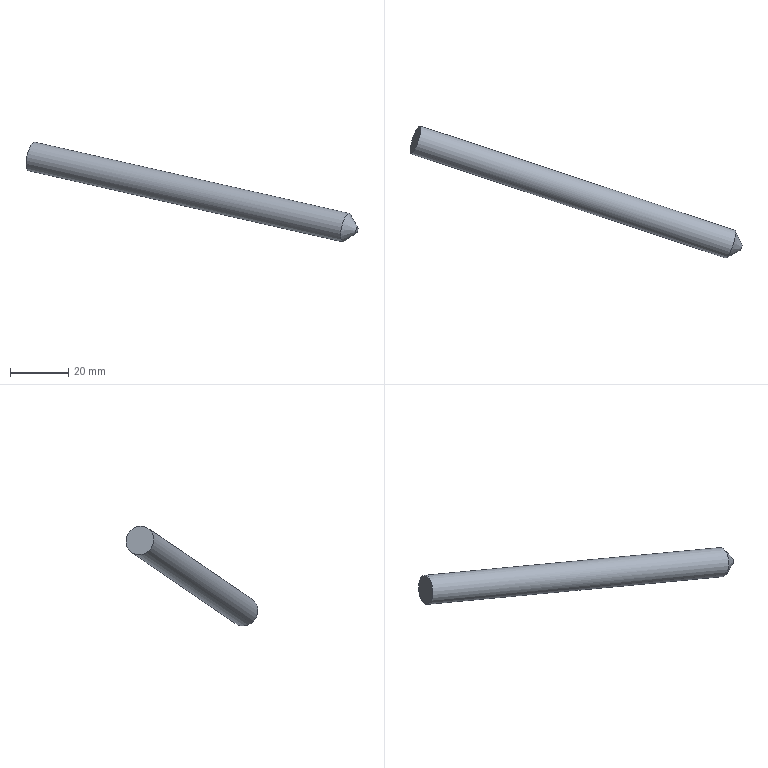Component | NX | PEN | 1 solid | 4 faces | box 113.61 x 45.15 x 34.15 mm | volume 9240 mm3 | plane 2 | cylinder 1 | cone 1 | commonest cylinder face diameters 10 x1
STEP:
#1=CARTESIAN_POINT('',(0.,0.,0.));
#2=DIRECTION('',(0.,0.,1.));
#3=DIRECTION('',(1.,0.,0.));
#4=AXIS2_PLACEMENT_3D('',#1,#2,#3);
#5=CARTESIAN_POINT('',(-47.005,-89.102,31.533));
#6=VERTEX_POINT('',#5);
#7=CARTESIAN_POINT('',(-46.915,-84.925,25.828));
#8=VERTEX_POINT('',#7);
#9=CARTESIAN_POINT('',(-48.275,-89.651,26.729));
#10=DIRECTION('',(-0.9282,0.3072,0.2101));
#11=DIRECTION('',(0.254,0.11,0.9609));
#12=AXIS2_PLACEMENT_3D('',#9,#10,#11);
#13=CIRCLE('',#12,5.);
#14=CARTESIAN_POINT('',(-44.562,-90.88,25.888));
#15=DIRECTION('',(-0.9282,0.3072,0.2101));
#16=DIRECTION('',(-0.254,-0.11,-0.9609));
#17=AXIS2_PLACEMENT_3D('',#14,#15,#16);
#18=CYLINDRICAL_SURFACE('',#17,5.);
#19=CARTESIAN_POINT('',(9.425,4.));
#20=DIRECTION('',(1.,0.));
#21=VECTOR('',#20,1.);
#22=LINE('',#19,#21);
#23=(GEOMETRIC_REPRESENTATION_CONTEXT(2)PARAMETRIC_REPRESENTATION_CONTEXT()REPRESENTATION_CONTEXT('',''));
#24=DEFINITIONAL_REPRESENTATION('',(#22),#23);
#25=PCURVE('',#18,#24);
#26=CARTESIAN_POINT('',(-44.562,-90.88,25.888));
#27=DIRECTION('',(-0.9282,0.3072,0.2101));
#28=DIRECTION('',(-0.254,-0.11,-0.9609));
#29=AXIS2_PLACEMENT_3D('',#26,#27,#28);
#30=CONICAL_SURFACE('',#29,1.,0.7854);
#31=CARTESIAN_POINT('',(3.142,4.));
#32=DIRECTION('',(1.,0.));
#33=VECTOR('',#32,1.);
#34=LINE('',#31,#33);
#35=(GEOMETRIC_REPRESENTATION_CONTEXT(2)PARAMETRIC_REPRESENTATION_CONTEXT()REPRESENTATION_CONTEXT('',''));
#36=DEFINITIONAL_REPRESENTATION('',(#34),#35);
#37=PCURVE('',#30,#36);
#38=SURFACE_CURVE('',#13,(#25,#37),.PCURVE_S1.);
#39=EDGE_CURVE('',#6,#8,#38,.T.);
#40=ORIENTED_EDGE('',*,*,#39,.T.);
#41=CARTESIAN_POINT('',(-154.581,-49.291,50.204));
#42=VERTEX_POINT('',#41);
#43=CARTESIAN_POINT('',(-46.915,-84.925,25.828));
#44=CARTESIAN_POINT('',(-154.581,-49.291,50.204));
#45=B_SPLINE_CURVE_WITH_KNOTS('',1,(#43,#44),.UNSPECIFIED.,.F.,.F.,(2,2),(4.,120.),.PIECEWISE_BEZIER_KNOTS.);
#46=CARTESIAN_POINT('',(10.996,0.));
#47=DIRECTION('',(0.,1.));
#48=VECTOR('',#47,1.);
#49=LINE('',#46,#48);
#50=(GEOMETRIC_REPRESENTATION_CONTEXT(2)PARAMETRIC_REPRESENTATION_CONTEXT()REPRESENTATION_CONTEXT('',''));
#51=DEFINITIONAL_REPRESENTATION('',(#49),#50);
#52=PCURVE('',#18,#51);
#53=CARTESIAN_POINT('',(4.712,0.));
#54=DIRECTION('',(0.,1.));
#55=VECTOR('',#54,1.);
#56=LINE('',#53,#55);
#57=(GEOMETRIC_REPRESENTATION_CONTEXT(2)PARAMETRIC_REPRESENTATION_CONTEXT()REPRESENTATION_CONTEXT('',''));
#58=DEFINITIONAL_REPRESENTATION('',(#56),#57);
#59=PCURVE('',#18,#58);
#60=SEAM_CURVE('',#45,(#52,#59),.PCURVE_S1.);
#61=EDGE_CURVE('',#8,#42,#60,.T.);
#62=ORIENTED_EDGE('',*,*,#61,.T.);
#63=CARTESIAN_POINT('',(-155.941,-54.017,51.104));
#64=DIRECTION('',(0.9282,-0.3072,-0.2101));
#65=DIRECTION('',(0.2721,0.9453,-0.1801));
#66=AXIS2_PLACEMENT_3D('',#63,#64,#65);
#67=CIRCLE('',#66,5.);
#68=CARTESIAN_POINT('',(10.996,120.));
#69=DIRECTION('',(-1.,0.));
#70=VECTOR('',#69,1.);
#71=LINE('',#68,#70);
#72=(GEOMETRIC_REPRESENTATION_CONTEXT(2)PARAMETRIC_REPRESENTATION_CONTEXT()REPRESENTATION_CONTEXT('',''));
#73=DEFINITIONAL_REPRESENTATION('',(#71),#72);
#74=PCURVE('',#18,#73);
#75=CARTESIAN_POINT('',(-155.941,-54.017,51.104));
#76=DIRECTION('',(0.9282,-0.3072,-0.2101));
#77=DIRECTION('',(0.254,0.11,0.9609));
#78=AXIS2_PLACEMENT_3D('',#75,#76,#77);
#79=PLANE('',#78);
#80=CARTESIAN_POINT('',(0.,0.));
#81=DIRECTION('',(0.,-1.));
#82=AXIS2_PLACEMENT_2D('',#80,#81);
#83=CIRCLE('',#82,5.);
#84=(GEOMETRIC_REPRESENTATION_CONTEXT(2)PARAMETRIC_REPRESENTATION_CONTEXT()REPRESENTATION_CONTEXT('',''));
#85=DEFINITIONAL_REPRESENTATION('',(#83),#84);
#86=PCURVE('',#79,#85);
#87=SURFACE_CURVE('',#67,(#74,#86),.PCURVE_S1.);
#88=EDGE_CURVE('',#42,#42,#87,.T.);
#89=ORIENTED_EDGE('',*,*,#88,.T.);
#90=ORIENTED_EDGE('',*,*,#61,.F.);
#91=CARTESIAN_POINT('',(-48.275,-89.651,26.729));
#92=DIRECTION('',(-0.9282,0.3072,0.2101));
#93=DIRECTION('',(0.254,0.11,0.9609));
#94=AXIS2_PLACEMENT_3D('',#91,#92,#93);
#95=CIRCLE('',#94,5.);
#96=CARTESIAN_POINT('',(3.142,4.));
#97=DIRECTION('',(1.,0.));
#98=VECTOR('',#97,1.);
#99=LINE('',#96,#98);
#100=(GEOMETRIC_REPRESENTATION_CONTEXT(2)PARAMETRIC_REPRESENTATION_CONTEXT()REPRESENTATION_CONTEXT('',''));
#101=DEFINITIONAL_REPRESENTATION('',(#99),#100);
#102=PCURVE('',#18,#101);
#103=CARTESIAN_POINT('',(3.142,4.));
#104=DIRECTION('',(1.,-0.));
#105=VECTOR('',#104,1.);
#106=LINE('',#103,#105);
#107=(GEOMETRIC_REPRESENTATION_CONTEXT(2)PARAMETRIC_REPRESENTATION_CONTEXT()REPRESENTATION_CONTEXT('',''));
#108=DEFINITIONAL_REPRESENTATION('',(#106),#107);
#109=PCURVE('',#30,#108);
#110=SURFACE_CURVE('',#95,(#102,#109),.PCURVE_S1.);
#111=EDGE_CURVE('',#8,#6,#110,.T.);
#112=ORIENTED_EDGE('',*,*,#111,.T.);
#113=EDGE_LOOP('',(#40,#62,#89,#90,#112));
#114=FACE_BOUND('',#113,.T.);
#115=ADVANCED_FACE('',(#114),#18,.T.);
#116=CARTESIAN_POINT('',(-44.308,-90.77,26.849));
#117=VERTEX_POINT('',#116);
#118=CARTESIAN_POINT('',(-44.562,-90.88,25.888));
#119=DIRECTION('',(0.9282,-0.3072,-0.2101));
#120=DIRECTION('',(0.254,0.11,0.9609));
#121=AXIS2_PLACEMENT_3D('',#118,#119,#120);
#122=CIRCLE('',#121,1.);
#123=CARTESIAN_POINT('',(-44.562,-90.88,25.888));
#124=DIRECTION('',(0.9282,-0.3072,-0.2101));
#125=DIRECTION('',(0.254,0.11,0.9609));
#126=AXIS2_PLACEMENT_3D('',#123,#124,#125);
#127=PLANE('',#126);
#128=CARTESIAN_POINT('',(0.,0.));
#129=DIRECTION('',(1.,0.));
#130=AXIS2_PLACEMENT_2D('',#128,#129);
#131=CIRCLE('',#130,1.);
#132=(GEOMETRIC_REPRESENTATION_CONTEXT(2)PARAMETRIC_REPRESENTATION_CONTEXT()REPRESENTATION_CONTEXT('',''));
#133=DEFINITIONAL_REPRESENTATION('',(#131),#132);
#134=PCURVE('',#127,#133);
#135=CARTESIAN_POINT('',(9.425,-0.));
#136=DIRECTION('',(-1.,0.));
#137=VECTOR('',#136,1.);
#138=LINE('',#135,#137);
#139=(GEOMETRIC_REPRESENTATION_CONTEXT(2)PARAMETRIC_REPRESENTATION_CONTEXT()REPRESENTATION_CONTEXT('',''));
#140=DEFINITIONAL_REPRESENTATION('',(#138),#139);
#141=PCURVE('',#30,#140);
#142=SURFACE_CURVE('',#122,(#134,#141),.PCURVE_S1.);
#143=EDGE_CURVE('',#117,#117,#142,.T.);
#144=ORIENTED_EDGE('',*,*,#143,.T.);
#145=EDGE_LOOP('',(#144));
#146=FACE_BOUND('',#145,.T.);
#147=ADVANCED_FACE('',(#146),#127,.T.);
#148=ORIENTED_EDGE('',*,*,#88,.F.);
#149=EDGE_LOOP('',(#148));
#150=FACE_BOUND('',#149,.T.);
#151=ADVANCED_FACE('',(#150),#79,.F.);
#152=ORIENTED_EDGE('',*,*,#39,.F.);
#153=CARTESIAN_POINT('',(-44.308,-90.77,26.849));
#154=CARTESIAN_POINT('',(-47.005,-89.102,31.533));
#155=B_SPLINE_CURVE_WITH_KNOTS('',1,(#153,#154),.UNSPECIFIED.,.F.,.F.,(2,2),(-0.,5.657),.PIECEWISE_BEZIER_KNOTS.);
#156=CARTESIAN_POINT('',(3.142,0.));
#157=DIRECTION('',(0.,1.));
#158=VECTOR('',#157,1.);
#159=LINE('',#156,#158);
#160=(GEOMETRIC_REPRESENTATION_CONTEXT(2)PARAMETRIC_REPRESENTATION_CONTEXT()REPRESENTATION_CONTEXT('',''));
#161=DEFINITIONAL_REPRESENTATION('',(#159),#160);
#162=PCURVE('',#30,#161);
#163=CARTESIAN_POINT('',(9.425,0.));
#164=DIRECTION('',(0.,1.));
#165=VECTOR('',#164,1.);
#166=LINE('',#163,#165);
#167=(GEOMETRIC_REPRESENTATION_CONTEXT(2)PARAMETRIC_REPRESENTATION_CONTEXT()REPRESENTATION_CONTEXT('',''));
#168=DEFINITIONAL_REPRESENTATION('',(#166),#167);
#169=PCURVE('',#30,#168);
#170=SEAM_CURVE('',#155,(#162,#169),.PCURVE_S1.);
#171=EDGE_CURVE('',#117,#6,#170,.T.);
#172=ORIENTED_EDGE('',*,*,#171,.F.);
#173=ORIENTED_EDGE('',*,*,#143,.F.);
#174=ORIENTED_EDGE('',*,*,#171,.T.);
#175=ORIENTED_EDGE('',*,*,#111,.F.);
#176=EDGE_LOOP('',(#152,#172,#173,#174,#175));
#177=FACE_BOUND('',#176,.T.);
#178=ADVANCED_FACE('',(#177),#30,.T.);
#179=CLOSED_SHELL('',(#115,#147,#151,#178));
#180=MANIFOLD_SOLID_BREP('',#179);
#181=(LENGTH_UNIT()NAMED_UNIT(*)SI_UNIT(.MILLI.,.METRE.));
#182=UNCERTAINTY_MEASURE_WITH_UNIT(LENGTH_MEASURE(0.00001),#181,'','');
#183=(NAMED_UNIT(*)PLANE_ANGLE_UNIT()SI_UNIT($,.RADIAN.));
#184=(NAMED_UNIT(*)SI_UNIT($,.STERADIAN.)SOLID_ANGLE_UNIT());
#185=(GEOMETRIC_REPRESENTATION_CONTEXT(3)GLOBAL_UNCERTAINTY_ASSIGNED_CONTEXT((#182))GLOBAL_UNIT_ASSIGNED_CONTEXT((#181,#183,#184))REPRESENTATION_CONTEXT('',''));
#186=ADVANCED_BREP_SHAPE_REPRESENTATION('',(#4,#180),#185);